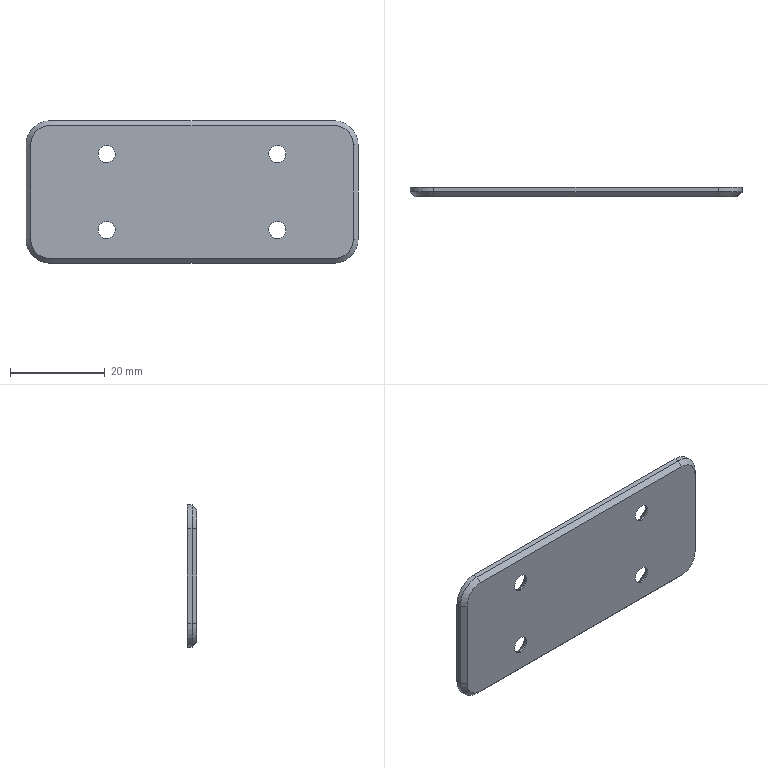CAM job | Mastercam | mm | 1 operations | part box 70 x 2 x 30
1. Surface Finish Flowline | 13 - 2-R0.5圆鼻铣刀